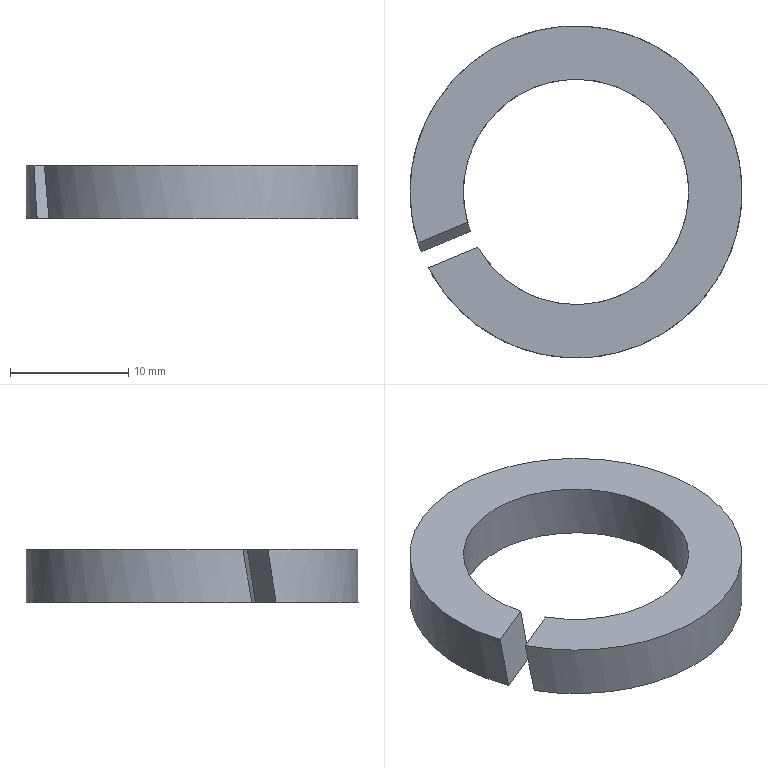Component | NX | GB93-87__18 | 1 solid | 6 faces | box 28.04 x 28.04 x 4.5 mm | volume 1451 mm3 | plane 4 | cylinder 2 | commonest cylinder face diameters 28.04 x1 19.04 x1
STEP:
#1=CARTESIAN_POINT('',(0.,0.,0.));
#2=DIRECTION('',(0.,0.,1.));
#3=DIRECTION('',(1.,0.,0.));
#4=AXIS2_PLACEMENT_3D('',#1,#2,#3);
#5=CARTESIAN_POINT('',(68.779,-123.057,-28.115));
#6=VERTEX_POINT('',#5);
#7=CARTESIAN_POINT('',(67.904,-120.947,-28.115));
#8=VERTEX_POINT('',#7);
#9=CARTESIAN_POINT('',(81.249,-116.649,-28.115));
#10=DIRECTION('',(0.,0.,1.));
#11=DIRECTION('',(0.9237,0.383,0.));
#12=AXIS2_PLACEMENT_3D('',#9,#10,#11);
#13=CIRCLE('',#12,14.02);
#14=CARTESIAN_POINT('',(81.249,-116.649,-28.115));
#15=DIRECTION('',(0.,0.,1.));
#16=DIRECTION('',(0.9237,0.383,0.));
#17=AXIS2_PLACEMENT_3D('',#14,#15,#16);
#18=CYLINDRICAL_SURFACE('',#17,14.02);
#19=CARTESIAN_POINT('',(-6.283,0.));
#20=DIRECTION('',(1.,0.));
#21=VECTOR('',#20,1.);
#22=LINE('',#19,#21);
#23=(GEOMETRIC_REPRESENTATION_CONTEXT(2)PARAMETRIC_REPRESENTATION_CONTEXT()REPRESENTATION_CONTEXT('',''));
#24=DEFINITIONAL_REPRESENTATION('',(#22),#23);
#25=PCURVE('',#18,#24);
#26=CARTESIAN_POINT('',(77.603,-107.855,-28.115));
#27=DIRECTION('',(0.,0.,1.));
#28=DIRECTION('',(0.9237,0.383,0.));
#29=AXIS2_PLACEMENT_3D('',#26,#27,#28);
#30=PLANE('',#29);
#31=CARTESIAN_POINT('',(0.,-9.52));
#32=DIRECTION('',(1.,0.));
#33=AXIS2_PLACEMENT_2D('',#31,#32);
#34=CIRCLE('',#33,14.02);
#35=(GEOMETRIC_REPRESENTATION_CONTEXT(2)PARAMETRIC_REPRESENTATION_CONTEXT()REPRESENTATION_CONTEXT('',''));
#36=DEFINITIONAL_REPRESENTATION('',(#34),#35);
#37=PCURVE('',#30,#36);
#38=SURFACE_CURVE('',#13,(#25,#37),.PCURVE_S1.);
#39=EDGE_CURVE('',#6,#8,#38,.T.);
#40=ORIENTED_EDGE('',*,*,#39,.F.);
#41=CARTESIAN_POINT('',(69.164,-123.756,-32.615));
#42=VERTEX_POINT('',#41);
#43=CARTESIAN_POINT('',(81.249,-116.649,-21.637));
#44=DIRECTION('',(0.3772,-0.9097,0.1736));
#45=DIRECTION('',(-0.06652,0.1604,0.9848));
#46=AXIS2_PLACEMENT_3D('',#43,#44,#45);
#47=ELLIPSE('',#46,80.738,14.02);
#48=CARTESIAN_POINT('',(-3.06,0.));
#49=CARTESIAN_POINT('',(-3.003,-4.5));
#50=B_SPLINE_CURVE_WITH_KNOTS('',1,(#48,#49),.UNSPECIFIED.,.F.,.F.,(2,2),(1.652,1.709),.PIECEWISE_BEZIER_KNOTS.);
#51=(GEOMETRIC_REPRESENTATION_CONTEXT(2)PARAMETRIC_REPRESENTATION_CONTEXT()REPRESENTATION_CONTEXT('',''));
#52=DEFINITIONAL_REPRESENTATION('',(#50),#51);
#53=PCURVE('',#18,#52);
#54=CARTESIAN_POINT('',(62.697,-126.811,-34.567));
#55=DIRECTION('',(-0.3772,0.9097,-0.1736));
#56=DIRECTION('',(0.06652,-0.1604,-0.9848));
#57=AXIS2_PLACEMENT_3D('',#54,#55,#56);
#58=PLANE('',#57);
#59=CARTESIAN_POINT('',(-93.868,-21.03));
#60=CARTESIAN_POINT('',(-93.868,3.253));
#61=CARTESIAN_POINT('',(27.239,-8.888));
#62=CARTESIAN_POINT('',(148.346,-21.03));
#63=CARTESIAN_POINT('',(27.239,-33.172));
#64=CARTESIAN_POINT('',(-93.868,-45.313));
#65=CARTESIAN_POINT('',(-93.868,-21.03));
#66=(BOUNDED_CURVE()B_SPLINE_CURVE(2,(#59,#60,#61,#62,#63,#64,#65),.UNSPECIFIED.,.T.,.F.)B_SPLINE_CURVE_WITH_KNOTS((1,2,2,2,2,1),(-2.094,0.,2.094,4.189,6.283,8.378),.UNSPECIFIED.)CURVE()GEOMETRIC_REPRESENTATION_ITEM()RATIONAL_B_SPLINE_CURVE((1.,0.5,1.,0.5,1.,0.5,1.))REPRESENTATION_ITEM(''));
#67=(GEOMETRIC_REPRESENTATION_CONTEXT(2)PARAMETRIC_REPRESENTATION_CONTEXT()REPRESENTATION_CONTEXT('',''));
#68=DEFINITIONAL_REPRESENTATION('',(#66),#67);
#69=PCURVE('',#58,#68);
#70=SURFACE_CURVE('',#47,(#53,#69),.PCURVE_S1.);
#71=EDGE_CURVE('',#6,#42,#70,.T.);
#72=ORIENTED_EDGE('',*,*,#71,.T.);
#73=CARTESIAN_POINT('',(68.169,-121.696,-32.615));
#74=VERTEX_POINT('',#73);
#75=CARTESIAN_POINT('',(81.249,-116.649,-32.615));
#76=DIRECTION('',(0.,0.,1.));
#77=DIRECTION('',(0.9237,0.383,0.));
#78=AXIS2_PLACEMENT_3D('',#75,#76,#77);
#79=CIRCLE('',#78,14.02);
#80=CARTESIAN_POINT('',(-6.283,-4.5));
#81=DIRECTION('',(1.,0.));
#82=VECTOR('',#81,1.);
#83=LINE('',#80,#82);
#84=(GEOMETRIC_REPRESENTATION_CONTEXT(2)PARAMETRIC_REPRESENTATION_CONTEXT()REPRESENTATION_CONTEXT('',''));
#85=DEFINITIONAL_REPRESENTATION('',(#83),#84);
#86=PCURVE('',#18,#85);
#87=CARTESIAN_POINT('',(75.879,-103.699,-32.615));
#88=DIRECTION('',(0.,0.,-1.));
#89=DIRECTION('',(-0.9237,-0.383,0.));
#90=AXIS2_PLACEMENT_3D('',#87,#88,#89);
#91=PLANE('',#90);
#92=CARTESIAN_POINT('',(-14.02,-14.02));
#93=CARTESIAN_POINT('',(-14.02,10.263));
#94=CARTESIAN_POINT('',(7.01,-1.878));
#95=CARTESIAN_POINT('',(28.04,-14.02));
#96=CARTESIAN_POINT('',(7.01,-26.162));
#97=CARTESIAN_POINT('',(-14.02,-38.303));
#98=CARTESIAN_POINT('',(-14.02,-14.02));
#99=(BOUNDED_CURVE()B_SPLINE_CURVE(2,(#92,#93,#94,#95,#96,#97,#98),.UNSPECIFIED.,.T.,.F.)B_SPLINE_CURVE_WITH_KNOTS((1,2,2,2,2,1),(-2.094,0.,2.094,4.189,6.283,8.378),.UNSPECIFIED.)CURVE()GEOMETRIC_REPRESENTATION_ITEM()RATIONAL_B_SPLINE_CURVE((1.,0.5,1.,0.5,1.,0.5,1.))REPRESENTATION_ITEM(''));
#100=(GEOMETRIC_REPRESENTATION_CONTEXT(2)PARAMETRIC_REPRESENTATION_CONTEXT()REPRESENTATION_CONTEXT('',''));
#101=DEFINITIONAL_REPRESENTATION('',(#99),#100);
#102=PCURVE('',#91,#101);
#103=SURFACE_CURVE('',#79,(#86,#102),.PCURVE_S1.);
#104=EDGE_CURVE('',#42,#74,#103,.T.);
#105=ORIENTED_EDGE('',*,*,#104,.T.);
#106=CARTESIAN_POINT('',(81.249,-116.649,-34.594));
#107=DIRECTION('',(-0.3772,0.9097,-0.1736));
#108=DIRECTION('',(-0.06652,0.1604,0.9848));
#109=AXIS2_PLACEMENT_3D('',#106,#107,#108);
#110=ELLIPSE('',#109,80.738,14.02);
#111=CARTESIAN_POINT('',(3.117,-4.5));
#112=CARTESIAN_POINT('',(3.06,0.));
#113=B_SPLINE_CURVE_WITH_KNOTS('',1,(#111,#112),.UNSPECIFIED.,.F.,.F.,(2,2),(4.737,4.794),.PIECEWISE_BEZIER_KNOTS.);
#114=(GEOMETRIC_REPRESENTATION_CONTEXT(2)PARAMETRIC_REPRESENTATION_CONTEXT()REPRESENTATION_CONTEXT('',''));
#115=DEFINITIONAL_REPRESENTATION('',(#113),#114);
#116=PCURVE('',#18,#115);
#117=CARTESIAN_POINT('',(60.95,-122.599,-21.663));
#118=DIRECTION('',(0.3772,-0.9097,0.1736));
#119=DIRECTION('',(-0.06652,0.1604,0.9848));
#120=AXIS2_PLACEMENT_3D('',#117,#118,#119);
#121=PLANE('',#120);
#122=CARTESIAN_POINT('',(67.608,-21.03));
#123=CARTESIAN_POINT('',(67.608,-45.313));
#124=CARTESIAN_POINT('',(-53.499,-33.172));
#125=CARTESIAN_POINT('',(-174.606,-21.03));
#126=CARTESIAN_POINT('',(-53.499,-8.888));
#127=CARTESIAN_POINT('',(67.608,3.253));
#128=CARTESIAN_POINT('',(67.608,-21.03));
#129=(BOUNDED_CURVE()B_SPLINE_CURVE(2,(#122,#123,#124,#125,#126,#127,#128),.UNSPECIFIED.,.T.,.F.)B_SPLINE_CURVE_WITH_KNOTS((1,2,2,2,2,1),(-2.094,0.,2.094,4.189,6.283,8.378),.UNSPECIFIED.)CURVE()GEOMETRIC_REPRESENTATION_ITEM()RATIONAL_B_SPLINE_CURVE((1.,0.5,1.,0.5,1.,0.5,1.))REPRESENTATION_ITEM(''));
#130=(GEOMETRIC_REPRESENTATION_CONTEXT(2)PARAMETRIC_REPRESENTATION_CONTEXT()REPRESENTATION_CONTEXT('',''));
#131=DEFINITIONAL_REPRESENTATION('',(#129),#130);
#132=PCURVE('',#121,#131);
#133=SURFACE_CURVE('',#110,(#116,#132),.PCURVE_S1.);
#134=EDGE_CURVE('',#74,#8,#133,.T.);
#135=ORIENTED_EDGE('',*,*,#134,.T.);
#136=EDGE_LOOP('',(#40,#72,#105,#135));
#137=FACE_BOUND('',#136,.T.);
#138=ADVANCED_FACE('',(#137),#18,.T.);
#139=ORIENTED_EDGE('',*,*,#104,.F.);
#140=CARTESIAN_POINT('',(73.381,-122.008,-32.615));
#141=VERTEX_POINT('',#140);
#142=CARTESIAN_POINT('',(81.991,-118.437,-32.615));
#143=DIRECTION('',(0.9237,0.383,0.));
#144=VECTOR('',#143,1.);
#145=LINE('',#142,#144);
#146=CARTESIAN_POINT('',(-0.,-15.956));
#147=DIRECTION('',(-1.,0.));
#148=VECTOR('',#147,1.);
#149=LINE('',#146,#148);
#150=(GEOMETRIC_REPRESENTATION_CONTEXT(2)PARAMETRIC_REPRESENTATION_CONTEXT()REPRESENTATION_CONTEXT('',''));
#151=DEFINITIONAL_REPRESENTATION('',(#149),#150);
#152=PCURVE('',#91,#151);
#153=CARTESIAN_POINT('',(-1.982,-21.03));
#154=DIRECTION('',(-0.,-1.));
#155=VECTOR('',#154,1.);
#156=LINE('',#153,#155);
#157=(GEOMETRIC_REPRESENTATION_CONTEXT(2)PARAMETRIC_REPRESENTATION_CONTEXT()REPRESENTATION_CONTEXT('',''));
#158=DEFINITIONAL_REPRESENTATION('',(#156),#157);
#159=PCURVE('',#58,#158);
#160=SURFACE_CURVE('',#145,(#152,#159),.PCURVE_S1.);
#161=EDGE_CURVE('',#42,#141,#160,.T.);
#162=ORIENTED_EDGE('',*,*,#161,.T.);
#163=CARTESIAN_POINT('',(72.328,-119.971,-32.615));
#164=VERTEX_POINT('',#163);
#165=CARTESIAN_POINT('',(81.249,-116.649,-32.615));
#166=DIRECTION('',(0.,0.,1.));
#167=DIRECTION('',(0.9237,0.383,0.));
#168=AXIS2_PLACEMENT_3D('',#165,#166,#167);
#169=CIRCLE('',#168,9.52);
#170=CARTESIAN_POINT('',(-9.52,-14.02));
#171=CARTESIAN_POINT('',(-9.52,2.469));
#172=CARTESIAN_POINT('',(4.76,-5.775));
#173=CARTESIAN_POINT('',(19.04,-14.02));
#174=CARTESIAN_POINT('',(4.76,-22.265));
#175=CARTESIAN_POINT('',(-9.52,-30.509));
#176=CARTESIAN_POINT('',(-9.52,-14.02));
#177=(BOUNDED_CURVE()B_SPLINE_CURVE(2,(#170,#171,#172,#173,#174,#175,#176),.UNSPECIFIED.,.T.,.F.)B_SPLINE_CURVE_WITH_KNOTS((1,2,2,2,2,1),(-2.094,0.,2.094,4.189,6.283,8.378),.UNSPECIFIED.)CURVE()GEOMETRIC_REPRESENTATION_ITEM()RATIONAL_B_SPLINE_CURVE((1.,0.5,1.,0.5,1.,0.5,1.))REPRESENTATION_ITEM(''));
#178=(GEOMETRIC_REPRESENTATION_CONTEXT(2)PARAMETRIC_REPRESENTATION_CONTEXT()REPRESENTATION_CONTEXT('',''));
#179=DEFINITIONAL_REPRESENTATION('',(#177),#178);
#180=PCURVE('',#91,#179);
#181=CARTESIAN_POINT('',(81.249,-116.649,-28.115));
#182=DIRECTION('',(0.,0.,1.));
#183=DIRECTION('',(0.9237,0.383,0.));
#184=AXIS2_PLACEMENT_3D('',#181,#182,#183);
#185=CYLINDRICAL_SURFACE('',#184,9.52);
#186=CARTESIAN_POINT('',(-6.283,-4.5));
#187=DIRECTION('',(1.,0.));
#188=VECTOR('',#187,1.);
#189=LINE('',#186,#188);
#190=(GEOMETRIC_REPRESENTATION_CONTEXT(2)PARAMETRIC_REPRESENTATION_CONTEXT()REPRESENTATION_CONTEXT('',''));
#191=DEFINITIONAL_REPRESENTATION('',(#189),#190);
#192=PCURVE('',#185,#191);
#193=SURFACE_CURVE('',#169,(#180,#192),.PCURVE_S1.);
#194=EDGE_CURVE('',#141,#164,#193,.T.);
#195=ORIENTED_EDGE('',*,*,#194,.T.);
#196=CARTESIAN_POINT('',(81.116,-116.327,-32.615));
#197=DIRECTION('',(-0.9237,-0.383,0.));
#198=VECTOR('',#197,1.);
#199=LINE('',#196,#198);
#200=CARTESIAN_POINT('',(-0.,-13.671));
#201=DIRECTION('',(1.,0.));
#202=VECTOR('',#201,1.);
#203=LINE('',#200,#202);
#204=(GEOMETRIC_REPRESENTATION_CONTEXT(2)PARAMETRIC_REPRESENTATION_CONTEXT()REPRESENTATION_CONTEXT('',''));
#205=DEFINITIONAL_REPRESENTATION('',(#203),#204);
#206=PCURVE('',#91,#205);
#207=CARTESIAN_POINT('',(-11.121,-21.03));
#208=DIRECTION('',(-0.,1.));
#209=VECTOR('',#208,1.);
#210=LINE('',#207,#209);
#211=(GEOMETRIC_REPRESENTATION_CONTEXT(2)PARAMETRIC_REPRESENTATION_CONTEXT()REPRESENTATION_CONTEXT('',''));
#212=DEFINITIONAL_REPRESENTATION('',(#210),#211);
#213=PCURVE('',#121,#212);
#214=SURFACE_CURVE('',#199,(#206,#213),.PCURVE_S1.);
#215=EDGE_CURVE('',#164,#74,#214,.T.);
#216=ORIENTED_EDGE('',*,*,#215,.T.);
#217=EDGE_LOOP('',(#139,#162,#195,#216));
#218=FACE_BOUND('',#217,.T.);
#219=ADVANCED_FACE('',(#218),#91,.T.);
#220=CARTESIAN_POINT('',(72.081,-119.214,-28.115));
#221=VERTEX_POINT('',#220);
#222=CARTESIAN_POINT('',(81.249,-116.649,-34.594));
#223=DIRECTION('',(0.3772,-0.9097,0.1736));
#224=DIRECTION('',(-0.06652,0.1604,0.9848));
#225=AXIS2_PLACEMENT_3D('',#222,#223,#224);
#226=ELLIPSE('',#225,54.823,9.52);
#227=CARTESIAN_POINT('',(3.021,0.));
#228=CARTESIAN_POINT('',(3.105,-4.5));
#229=B_SPLINE_CURVE_WITH_KNOTS('',1,(#227,#228),.UNSPECIFIED.,.F.,.F.,(2,2),(1.451,1.534),.PIECEWISE_BEZIER_KNOTS.);
#230=(GEOMETRIC_REPRESENTATION_CONTEXT(2)PARAMETRIC_REPRESENTATION_CONTEXT()REPRESENTATION_CONTEXT('',''));
#231=DEFINITIONAL_REPRESENTATION('',(#229),#230);
#232=PCURVE('',#185,#231);
#233=CARTESIAN_POINT('',(-13.13,-21.03));
#234=DIRECTION('',(1.,-0.));
#235=AXIS2_PLACEMENT_2D('',#233,#234);
#236=ELLIPSE('',#235,54.823,9.52);
#237=(GEOMETRIC_REPRESENTATION_CONTEXT(2)PARAMETRIC_REPRESENTATION_CONTEXT()REPRESENTATION_CONTEXT('',''));
#238=DEFINITIONAL_REPRESENTATION('',(#236),#237);
#239=PCURVE('',#121,#238);
#240=SURFACE_CURVE('',#226,(#232,#239),.PCURVE_S1.);
#241=EDGE_CURVE('',#221,#164,#240,.T.);
#242=ORIENTED_EDGE('',*,*,#241,.F.);
#243=CARTESIAN_POINT('',(72.957,-121.325,-28.115));
#244=VERTEX_POINT('',#243);
#245=CARTESIAN_POINT('',(81.249,-116.649,-28.115));
#246=DIRECTION('',(0.,0.,1.));
#247=DIRECTION('',(0.9237,0.383,0.));
#248=AXIS2_PLACEMENT_3D('',#245,#246,#247);
#249=CIRCLE('',#248,9.52);
#250=CARTESIAN_POINT('',(-6.283,0.));
#251=DIRECTION('',(1.,0.));
#252=VECTOR('',#251,1.);
#253=LINE('',#250,#252);
#254=(GEOMETRIC_REPRESENTATION_CONTEXT(2)PARAMETRIC_REPRESENTATION_CONTEXT()REPRESENTATION_CONTEXT('',''));
#255=DEFINITIONAL_REPRESENTATION('',(#253),#254);
#256=PCURVE('',#185,#255);
#257=CARTESIAN_POINT('',(0.,-9.52));
#258=DIRECTION('',(1.,0.));
#259=AXIS2_PLACEMENT_2D('',#257,#258);
#260=CIRCLE('',#259,9.52);
#261=(GEOMETRIC_REPRESENTATION_CONTEXT(2)PARAMETRIC_REPRESENTATION_CONTEXT()REPRESENTATION_CONTEXT('',''));
#262=DEFINITIONAL_REPRESENTATION('',(#260),#261);
#263=PCURVE('',#30,#262);
#264=SURFACE_CURVE('',#249,(#256,#263),.PCURVE_S1.);
#265=EDGE_CURVE('',#244,#221,#264,.T.);
#266=ORIENTED_EDGE('',*,*,#265,.F.);
#267=CARTESIAN_POINT('',(81.249,-116.649,-21.637));
#268=DIRECTION('',(-0.3772,0.9097,-0.1736));
#269=DIRECTION('',(-0.06652,0.1604,0.9848));
#270=AXIS2_PLACEMENT_3D('',#267,#268,#269);
#271=ELLIPSE('',#270,54.823,9.52);
#272=CARTESIAN_POINT('',(-2.937,-4.5));
#273=CARTESIAN_POINT('',(-3.021,0.));
#274=B_SPLINE_CURVE_WITH_KNOTS('',1,(#272,#273),.UNSPECIFIED.,.F.,.F.,(2,2),(4.508,4.592),.PIECEWISE_BEZIER_KNOTS.);
#275=(GEOMETRIC_REPRESENTATION_CONTEXT(2)PARAMETRIC_REPRESENTATION_CONTEXT()REPRESENTATION_CONTEXT('',''));
#276=DEFINITIONAL_REPRESENTATION('',(#274),#275);
#277=PCURVE('',#185,#276);
#278=CARTESIAN_POINT('',(-13.13,-21.03));
#279=DIRECTION('',(-1.,-0.));
#280=AXIS2_PLACEMENT_2D('',#278,#279);
#281=ELLIPSE('',#280,54.823,9.52);
#282=(GEOMETRIC_REPRESENTATION_CONTEXT(2)PARAMETRIC_REPRESENTATION_CONTEXT()REPRESENTATION_CONTEXT('',''));
#283=DEFINITIONAL_REPRESENTATION('',(#281),#282);
#284=PCURVE('',#58,#283);
#285=SURFACE_CURVE('',#271,(#277,#284),.PCURVE_S1.);
#286=EDGE_CURVE('',#141,#244,#285,.T.);
#287=ORIENTED_EDGE('',*,*,#286,.F.);
#288=ORIENTED_EDGE('',*,*,#194,.T.);
#289=EDGE_LOOP('',(#242,#266,#287,#288));
#290=FACE_BOUND('',#289,.F.);
#291=ADVANCED_FACE('',(#290),#185,.F.);
#292=ORIENTED_EDGE('',*,*,#265,.F.);
#293=CARTESIAN_POINT('',(81.687,-117.704,-28.115));
#294=DIRECTION('',(-0.9237,-0.383,0.));
#295=VECTOR('',#294,1.);
#296=LINE('',#293,#295);
#297=CARTESIAN_POINT('',(0.,-10.662));
#298=DIRECTION('',(-1.,0.));
#299=VECTOR('',#298,1.);
#300=LINE('',#297,#299);
#301=(GEOMETRIC_REPRESENTATION_CONTEXT(2)PARAMETRIC_REPRESENTATION_CONTEXT()REPRESENTATION_CONTEXT('',''));
#302=DEFINITIONAL_REPRESENTATION('',(#300),#301);
#303=PCURVE('',#30,#302);
#304=CARTESIAN_POINT('',(-6.552,-21.03));
#305=DIRECTION('',(0.,1.));
#306=VECTOR('',#305,1.);
#307=LINE('',#304,#306);
#308=(GEOMETRIC_REPRESENTATION_CONTEXT(2)PARAMETRIC_REPRESENTATION_CONTEXT()REPRESENTATION_CONTEXT('',''));
#309=DEFINITIONAL_REPRESENTATION('',(#307),#308);
#310=PCURVE('',#58,#309);
#311=SURFACE_CURVE('',#296,(#303,#310),.PCURVE_S1.);
#312=EDGE_CURVE('',#244,#6,#311,.T.);
#313=ORIENTED_EDGE('',*,*,#312,.T.);
#314=ORIENTED_EDGE('',*,*,#39,.T.);
#315=CARTESIAN_POINT('',(80.812,-115.594,-28.115));
#316=DIRECTION('',(0.9237,0.383,0.));
#317=VECTOR('',#316,1.);
#318=LINE('',#315,#317);
#319=CARTESIAN_POINT('',(0.,-8.378));
#320=DIRECTION('',(1.,0.));
#321=VECTOR('',#320,1.);
#322=LINE('',#319,#321);
#323=(GEOMETRIC_REPRESENTATION_CONTEXT(2)PARAMETRIC_REPRESENTATION_CONTEXT()REPRESENTATION_CONTEXT('',''));
#324=DEFINITIONAL_REPRESENTATION('',(#322),#323);
#325=PCURVE('',#30,#324);
#326=CARTESIAN_POINT('',(-6.552,-21.03));
#327=DIRECTION('',(0.,-1.));
#328=VECTOR('',#327,1.);
#329=LINE('',#326,#328);
#330=(GEOMETRIC_REPRESENTATION_CONTEXT(2)PARAMETRIC_REPRESENTATION_CONTEXT()REPRESENTATION_CONTEXT('',''));
#331=DEFINITIONAL_REPRESENTATION('',(#329),#330);
#332=PCURVE('',#121,#331);
#333=SURFACE_CURVE('',#318,(#325,#332),.PCURVE_S1.);
#334=EDGE_CURVE('',#8,#221,#333,.T.);
#335=ORIENTED_EDGE('',*,*,#334,.T.);
#336=EDGE_LOOP('',(#292,#313,#314,#335));
#337=FACE_BOUND('',#336,.T.);
#338=ADVANCED_FACE('',(#337),#30,.T.);
#339=ORIENTED_EDGE('',*,*,#215,.F.);
#340=ORIENTED_EDGE('',*,*,#241,.F.);
#341=ORIENTED_EDGE('',*,*,#334,.F.);
#342=ORIENTED_EDGE('',*,*,#134,.F.);
#343=EDGE_LOOP('',(#339,#340,#341,#342));
#344=FACE_BOUND('',#343,.T.);
#345=ADVANCED_FACE('',(#344),#121,.T.);
#346=ORIENTED_EDGE('',*,*,#312,.F.);
#347=ORIENTED_EDGE('',*,*,#286,.F.);
#348=ORIENTED_EDGE('',*,*,#161,.F.);
#349=ORIENTED_EDGE('',*,*,#71,.F.);
#350=EDGE_LOOP('',(#346,#347,#348,#349));
#351=FACE_BOUND('',#350,.T.);
#352=ADVANCED_FACE('',(#351),#58,.T.);
#353=CLOSED_SHELL('',(#138,#219,#291,#338,#345,#352));
#354=MANIFOLD_SOLID_BREP('',#353);
#355=(LENGTH_UNIT()NAMED_UNIT(*)SI_UNIT(.MILLI.,.METRE.));
#356=UNCERTAINTY_MEASURE_WITH_UNIT(LENGTH_MEASURE(0.002),#355,'','');
#357=(NAMED_UNIT(*)PLANE_ANGLE_UNIT()SI_UNIT($,.RADIAN.));
#358=(NAMED_UNIT(*)SI_UNIT($,.STERADIAN.)SOLID_ANGLE_UNIT());
#359=(GEOMETRIC_REPRESENTATION_CONTEXT(3)GLOBAL_UNCERTAINTY_ASSIGNED_CONTEXT((#356))GLOBAL_UNIT_ASSIGNED_CONTEXT((#355,#357,#358))REPRESENTATION_CONTEXT('',''));
#360=ADVANCED_BREP_SHAPE_REPRESENTATION('',(#4,#354),#359);